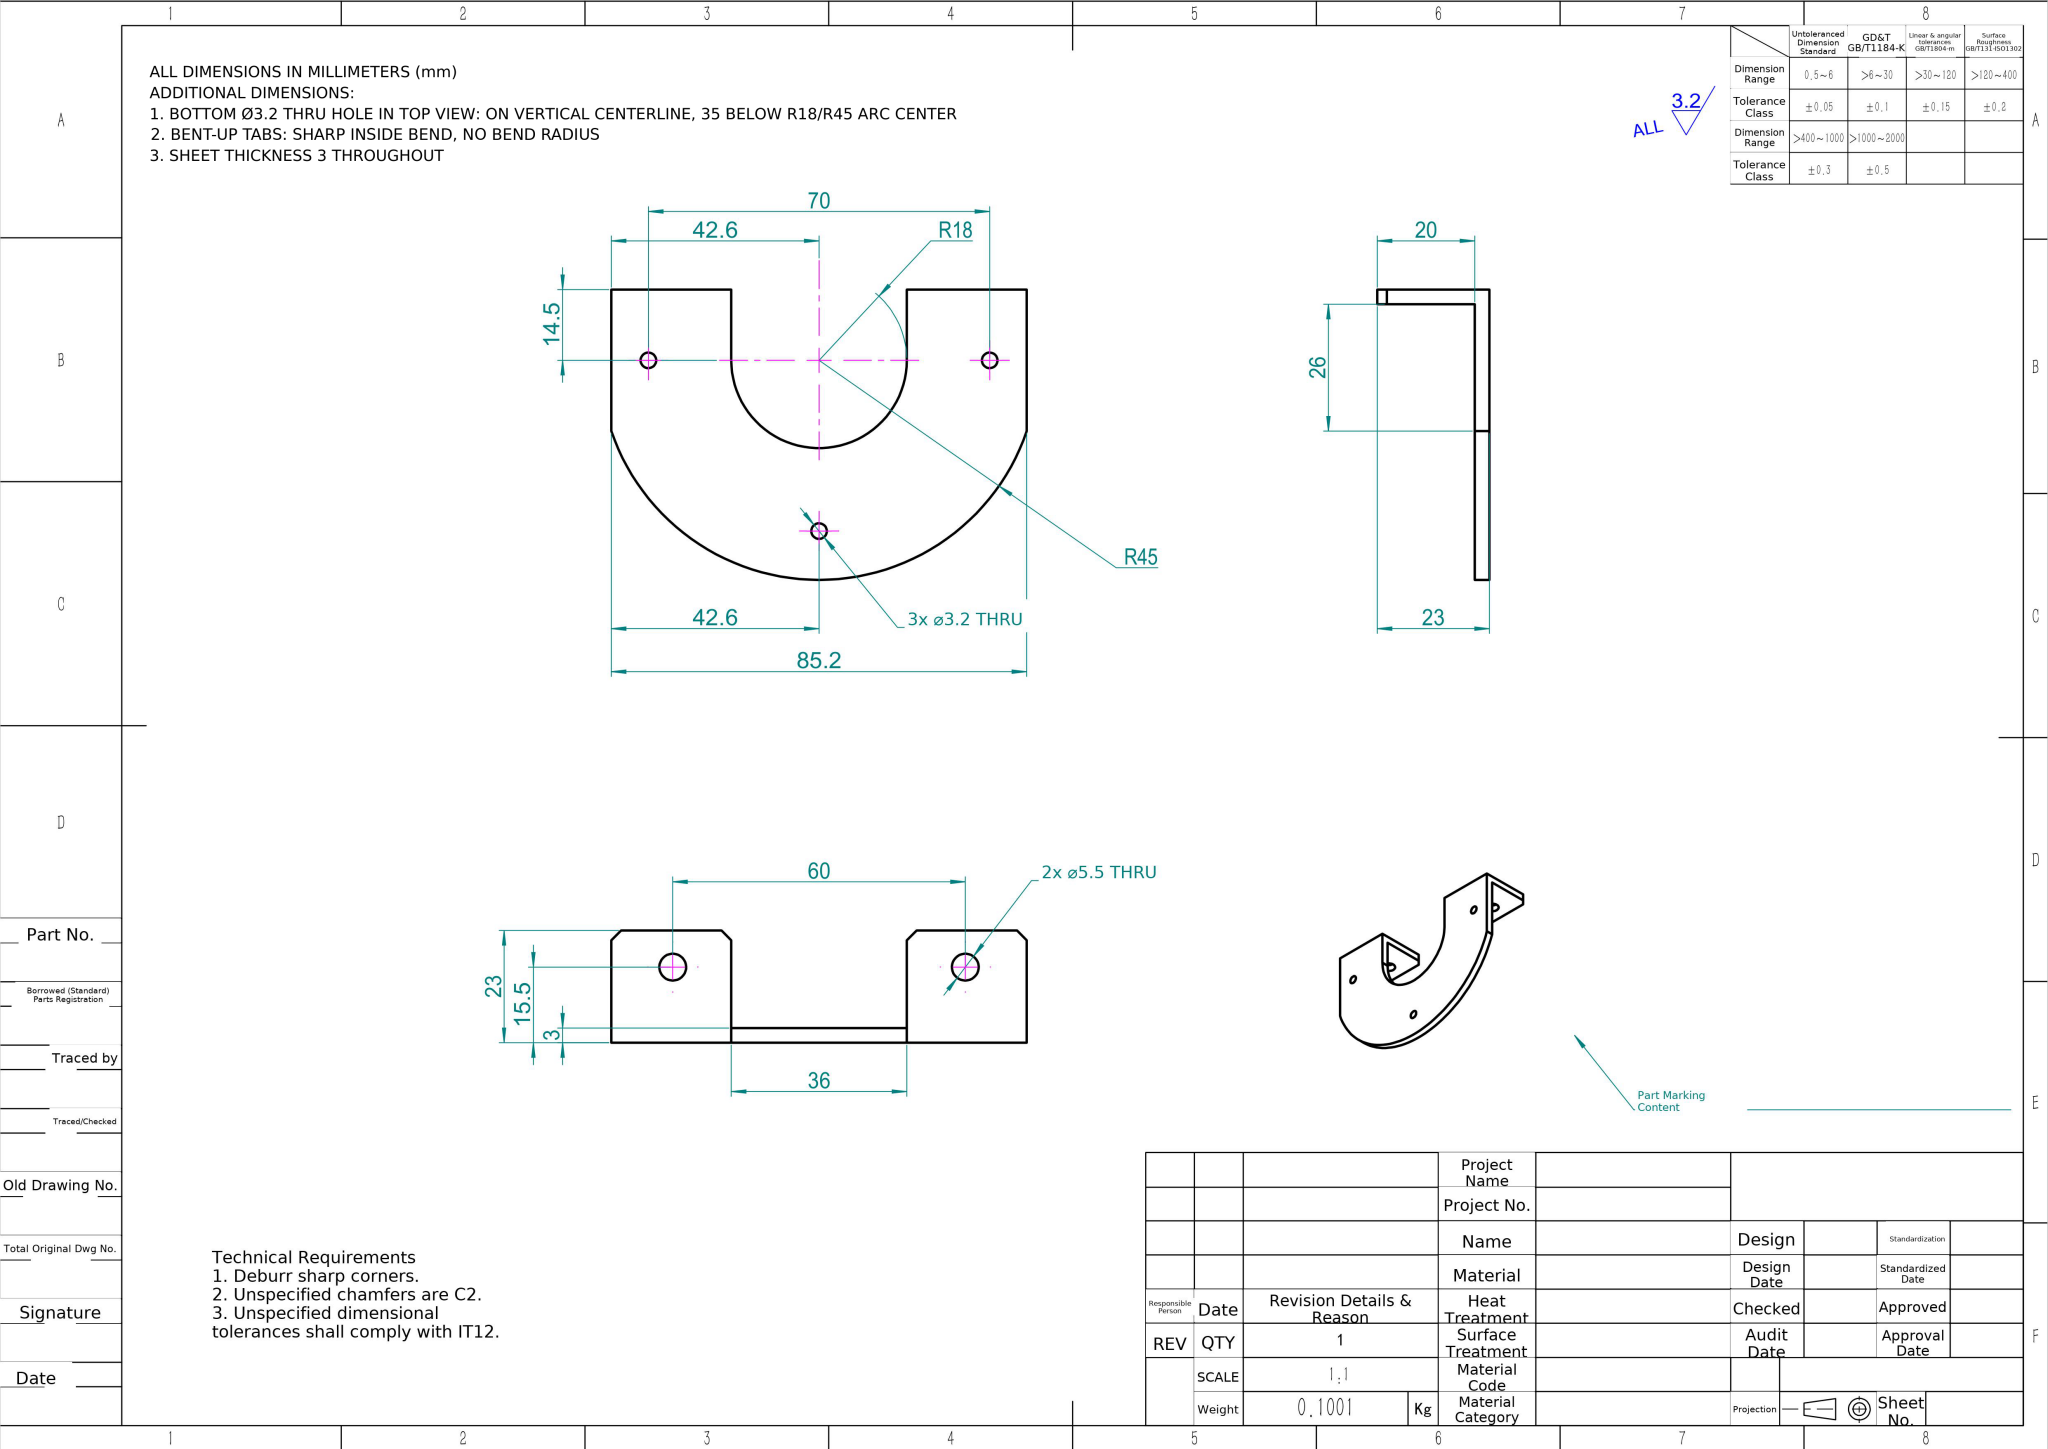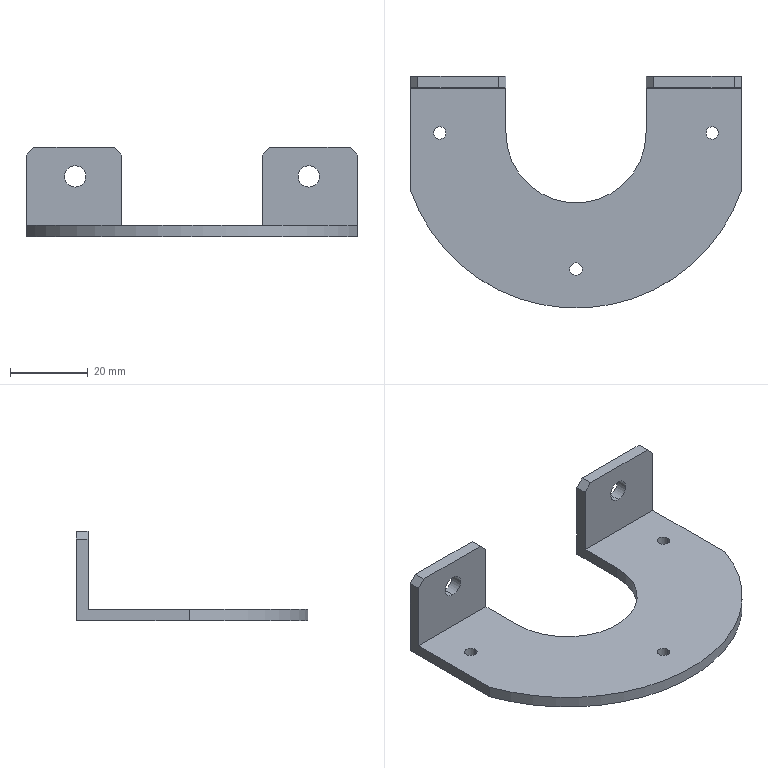Part | NX | mm | 1 solid | 28 faces | box 85.2 x 59.5 x 23 mm | volume 12729 mm3 | plane 16 | cylinder 12 | commonest cylinder face diameters 3.2 x6 5.5 x4 90 x1 36 x1
STEP:
#1=CARTESIAN_POINT('',(-36.6,0.,-0.));
#2=VERTEX_POINT('',#1);
#3=CARTESIAN_POINT('',(-33.4,0.,-0.));
#4=VERTEX_POINT('',#3);
#5=CARTESIAN_POINT('',(-35.,0.,-0.));
#6=DIRECTION('',(-0.,-0.,1.));
#7=DIRECTION('',(1.,0.,0.));
#8=AXIS2_PLACEMENT_3D('',#5,#6,#7);
#9=CIRCLE('',#8,1.6);
#10=EDGE_CURVE('',#2,#4,#9,.T.);
#11=ORIENTED_EDGE('',*,*,#10,.F.);
#12=CARTESIAN_POINT('',(-36.6,0.,3.));
#13=VERTEX_POINT('',#12);
#14=CARTESIAN_POINT('',(-36.6,0.,-0.));
#15=DIRECTION('',(-0.,-0.,1.));
#16=VECTOR('',#15,1000.);
#17=LINE('',#14,#16);
#18=EDGE_CURVE('',#2,#13,#17,.T.);
#19=ORIENTED_EDGE('',*,*,#18,.T.);
#20=CARTESIAN_POINT('',(-33.4,0.,3.));
#21=VERTEX_POINT('',#20);
#22=CARTESIAN_POINT('',(-35.,0.,3.));
#23=DIRECTION('',(-0.,-0.,1.));
#24=DIRECTION('',(1.,0.,0.));
#25=AXIS2_PLACEMENT_3D('',#22,#23,#24);
#26=CIRCLE('',#25,1.6);
#27=EDGE_CURVE('',#13,#21,#26,.T.);
#28=ORIENTED_EDGE('',*,*,#27,.T.);
#29=CARTESIAN_POINT('',(-33.4,0.,-0.));
#30=DIRECTION('',(-0.,-0.,1.));
#31=VECTOR('',#30,1000.);
#32=LINE('',#29,#31);
#33=EDGE_CURVE('',#4,#21,#32,.T.);
#34=ORIENTED_EDGE('',*,*,#33,.F.);
#35=EDGE_LOOP('',(#11,#19,#28,#34));
#36=FACE_OUTER_BOUND('',#35,.T.);
#37=CARTESIAN_POINT('',(-35.,0.,-0.));
#38=DIRECTION('',(-0.,-0.,1.));
#39=DIRECTION('',(1.,0.,0.));
#40=AXIS2_PLACEMENT_3D('',#37,#38,#39);
#41=CYLINDRICAL_SURFACE('',#40,1.6);
#42=ADVANCED_FACE('',(#36),#41,.F.);
#43=CARTESIAN_POINT('',(-1.6,-35.,-0.));
#44=VERTEX_POINT('',#43);
#45=CARTESIAN_POINT('',(1.6,-35.,0.));
#46=VERTEX_POINT('',#45);
#47=CARTESIAN_POINT('',(0.,-35.,0.));
#48=DIRECTION('',(-0.,-0.,1.));
#49=DIRECTION('',(1.,0.,0.));
#50=AXIS2_PLACEMENT_3D('',#47,#48,#49);
#51=CIRCLE('',#50,1.6);
#52=EDGE_CURVE('',#44,#46,#51,.T.);
#53=ORIENTED_EDGE('',*,*,#52,.F.);
#54=CARTESIAN_POINT('',(-1.6,-35.,3.));
#55=VERTEX_POINT('',#54);
#56=CARTESIAN_POINT('',(-1.6,-35.,-0.));
#57=DIRECTION('',(-0.,-0.,1.));
#58=VECTOR('',#57,1000.);
#59=LINE('',#56,#58);
#60=EDGE_CURVE('',#44,#55,#59,.T.);
#61=ORIENTED_EDGE('',*,*,#60,.T.);
#62=CARTESIAN_POINT('',(1.6,-35.,3.));
#63=VERTEX_POINT('',#62);
#64=CARTESIAN_POINT('',(-0.,-35.,3.));
#65=DIRECTION('',(-0.,-0.,1.));
#66=DIRECTION('',(1.,0.,0.));
#67=AXIS2_PLACEMENT_3D('',#64,#65,#66);
#68=CIRCLE('',#67,1.6);
#69=EDGE_CURVE('',#55,#63,#68,.T.);
#70=ORIENTED_EDGE('',*,*,#69,.T.);
#71=CARTESIAN_POINT('',(1.6,-35.,0.));
#72=DIRECTION('',(-0.,-0.,1.));
#73=VECTOR('',#72,1000.);
#74=LINE('',#71,#73);
#75=EDGE_CURVE('',#46,#63,#74,.T.);
#76=ORIENTED_EDGE('',*,*,#75,.F.);
#77=EDGE_LOOP('',(#53,#61,#70,#76));
#78=FACE_OUTER_BOUND('',#77,.T.);
#79=CARTESIAN_POINT('',(0.,-35.,0.));
#80=DIRECTION('',(-0.,-0.,1.));
#81=DIRECTION('',(1.,0.,0.));
#82=AXIS2_PLACEMENT_3D('',#79,#80,#81);
#83=CYLINDRICAL_SURFACE('',#82,1.6);
#84=ADVANCED_FACE('',(#78),#83,.F.);
#85=CARTESIAN_POINT('',(33.4,0.,-0.));
#86=VERTEX_POINT('',#85);
#87=CARTESIAN_POINT('',(36.6,0.,-0.));
#88=VERTEX_POINT('',#87);
#89=CARTESIAN_POINT('',(35.,0.,-0.));
#90=DIRECTION('',(-0.,-0.,1.));
#91=DIRECTION('',(1.,0.,0.));
#92=AXIS2_PLACEMENT_3D('',#89,#90,#91);
#93=CIRCLE('',#92,1.6);
#94=EDGE_CURVE('',#86,#88,#93,.T.);
#95=ORIENTED_EDGE('',*,*,#94,.F.);
#96=CARTESIAN_POINT('',(33.4,0.,3.));
#97=VERTEX_POINT('',#96);
#98=CARTESIAN_POINT('',(33.4,0.,-0.));
#99=DIRECTION('',(-0.,-0.,1.));
#100=VECTOR('',#99,1000.);
#101=LINE('',#98,#100);
#102=EDGE_CURVE('',#86,#97,#101,.T.);
#103=ORIENTED_EDGE('',*,*,#102,.T.);
#104=CARTESIAN_POINT('',(36.6,0.,3.));
#105=VERTEX_POINT('',#104);
#106=CARTESIAN_POINT('',(35.,0.,3.));
#107=DIRECTION('',(-0.,-0.,1.));
#108=DIRECTION('',(1.,0.,0.));
#109=AXIS2_PLACEMENT_3D('',#106,#107,#108);
#110=CIRCLE('',#109,1.6);
#111=EDGE_CURVE('',#97,#105,#110,.T.);
#112=ORIENTED_EDGE('',*,*,#111,.T.);
#113=CARTESIAN_POINT('',(36.6,0.,-0.));
#114=DIRECTION('',(-0.,-0.,1.));
#115=VECTOR('',#114,1000.);
#116=LINE('',#113,#115);
#117=EDGE_CURVE('',#88,#105,#116,.T.);
#118=ORIENTED_EDGE('',*,*,#117,.F.);
#119=EDGE_LOOP('',(#95,#103,#112,#118));
#120=FACE_OUTER_BOUND('',#119,.T.);
#121=CARTESIAN_POINT('',(35.,0.,-0.));
#122=DIRECTION('',(-0.,-0.,1.));
#123=DIRECTION('',(1.,0.,0.));
#124=AXIS2_PLACEMENT_3D('',#121,#122,#123);
#125=CYLINDRICAL_SURFACE('',#124,1.6);
#126=ADVANCED_FACE('',(#120),#125,.F.);
#127=CARTESIAN_POINT('',(-30.,14.5,18.25));
#128=VERTEX_POINT('',#127);
#129=CARTESIAN_POINT('',(-30.,14.5,12.75));
#130=VERTEX_POINT('',#129);
#131=CARTESIAN_POINT('',(-30.,14.5,15.5));
#132=DIRECTION('',(-0.,-1.,0.));
#133=DIRECTION('',(0.,0.,-1.));
#134=AXIS2_PLACEMENT_3D('',#131,#132,#133);
#135=CIRCLE('',#134,2.75);
#136=EDGE_CURVE('',#128,#130,#135,.T.);
#137=ORIENTED_EDGE('',*,*,#136,.F.);
#138=CARTESIAN_POINT('',(-30.,11.5,18.25));
#139=VERTEX_POINT('',#138);
#140=CARTESIAN_POINT('',(-30.,14.5,18.25));
#141=DIRECTION('',(-0.,-1.,0.));
#142=VECTOR('',#141,1000.);
#143=LINE('',#140,#142);
#144=EDGE_CURVE('',#128,#139,#143,.T.);
#145=ORIENTED_EDGE('',*,*,#144,.T.);
#146=CARTESIAN_POINT('',(-30.,11.5,12.75));
#147=VERTEX_POINT('',#146);
#148=CARTESIAN_POINT('',(-30.,11.5,15.5));
#149=DIRECTION('',(-0.,-1.,0.));
#150=DIRECTION('',(0.,0.,-1.));
#151=AXIS2_PLACEMENT_3D('',#148,#149,#150);
#152=CIRCLE('',#151,2.75);
#153=EDGE_CURVE('',#139,#147,#152,.T.);
#154=ORIENTED_EDGE('',*,*,#153,.T.);
#155=CARTESIAN_POINT('',(-30.,14.5,12.75));
#156=DIRECTION('',(-0.,-1.,0.));
#157=VECTOR('',#156,1000.);
#158=LINE('',#155,#157);
#159=EDGE_CURVE('',#130,#147,#158,.T.);
#160=ORIENTED_EDGE('',*,*,#159,.F.);
#161=EDGE_LOOP('',(#137,#145,#154,#160));
#162=FACE_OUTER_BOUND('',#161,.T.);
#163=CARTESIAN_POINT('',(-30.,14.5,15.5));
#164=DIRECTION('',(-0.,-1.,0.));
#165=DIRECTION('',(0.,0.,-1.));
#166=AXIS2_PLACEMENT_3D('',#163,#164,#165);
#167=CYLINDRICAL_SURFACE('',#166,2.75);
#168=ADVANCED_FACE('',(#162),#167,.F.);
#169=CARTESIAN_POINT('',(30.,14.5,18.25));
#170=VERTEX_POINT('',#169);
#171=CARTESIAN_POINT('',(30.,14.5,12.75));
#172=VERTEX_POINT('',#171);
#173=CARTESIAN_POINT('',(30.,14.5,15.5));
#174=DIRECTION('',(-0.,-1.,0.));
#175=DIRECTION('',(0.,0.,-1.));
#176=AXIS2_PLACEMENT_3D('',#173,#174,#175);
#177=CIRCLE('',#176,2.75);
#178=EDGE_CURVE('',#170,#172,#177,.T.);
#179=ORIENTED_EDGE('',*,*,#178,.F.);
#180=CARTESIAN_POINT('',(30.,11.5,18.25));
#181=VERTEX_POINT('',#180);
#182=CARTESIAN_POINT('',(30.,14.5,18.25));
#183=DIRECTION('',(-0.,-1.,0.));
#184=VECTOR('',#183,1000.);
#185=LINE('',#182,#184);
#186=EDGE_CURVE('',#170,#181,#185,.T.);
#187=ORIENTED_EDGE('',*,*,#186,.T.);
#188=CARTESIAN_POINT('',(30.,11.5,12.75));
#189=VERTEX_POINT('',#188);
#190=CARTESIAN_POINT('',(30.,11.5,15.5));
#191=DIRECTION('',(-0.,-1.,0.));
#192=DIRECTION('',(0.,0.,-1.));
#193=AXIS2_PLACEMENT_3D('',#190,#191,#192);
#194=CIRCLE('',#193,2.75);
#195=EDGE_CURVE('',#181,#189,#194,.T.);
#196=ORIENTED_EDGE('',*,*,#195,.T.);
#197=CARTESIAN_POINT('',(30.,14.5,12.75));
#198=DIRECTION('',(-0.,-1.,0.));
#199=VECTOR('',#198,1000.);
#200=LINE('',#197,#199);
#201=EDGE_CURVE('',#172,#189,#200,.T.);
#202=ORIENTED_EDGE('',*,*,#201,.F.);
#203=EDGE_LOOP('',(#179,#187,#196,#202));
#204=FACE_OUTER_BOUND('',#203,.T.);
#205=CARTESIAN_POINT('',(30.,14.5,15.5));
#206=DIRECTION('',(-0.,-1.,0.));
#207=DIRECTION('',(0.,0.,-1.));
#208=AXIS2_PLACEMENT_3D('',#205,#206,#207);
#209=CYLINDRICAL_SURFACE('',#208,2.75);
#210=ADVANCED_FACE('',(#204),#209,.F.);
#211=CARTESIAN_POINT('',(-35.,0.,3.));
#212=DIRECTION('',(-0.,-0.,1.));
#213=DIRECTION('',(1.,0.,0.));
#214=AXIS2_PLACEMENT_3D('',#211,#212,#213);
#215=CIRCLE('',#214,1.6);
#216=EDGE_CURVE('',#21,#13,#215,.T.);
#217=ORIENTED_EDGE('',*,*,#216,.F.);
#218=ORIENTED_EDGE('',*,*,#27,.F.);
#219=EDGE_LOOP('',(#217,#218));
#220=FACE_BOUND('',#219,.T.);
#221=CARTESIAN_POINT('',(-0.,-35.,3.));
#222=DIRECTION('',(-0.,-0.,1.));
#223=DIRECTION('',(1.,0.,0.));
#224=AXIS2_PLACEMENT_3D('',#221,#222,#223);
#225=CIRCLE('',#224,1.6);
#226=EDGE_CURVE('',#63,#55,#225,.T.);
#227=ORIENTED_EDGE('',*,*,#226,.F.);
#228=ORIENTED_EDGE('',*,*,#69,.F.);
#229=EDGE_LOOP('',(#227,#228));
#230=FACE_BOUND('',#229,.T.);
#231=CARTESIAN_POINT('',(35.,0.,3.));
#232=DIRECTION('',(-0.,-0.,1.));
#233=DIRECTION('',(1.,0.,0.));
#234=AXIS2_PLACEMENT_3D('',#231,#232,#233);
#235=CIRCLE('',#234,1.6);
#236=EDGE_CURVE('',#105,#97,#235,.T.);
#237=ORIENTED_EDGE('',*,*,#236,.F.);
#238=ORIENTED_EDGE('',*,*,#111,.F.);
#239=EDGE_LOOP('',(#237,#238));
#240=FACE_BOUND('',#239,.T.);
#241=CARTESIAN_POINT('',(-42.6,11.5,3.));
#242=VERTEX_POINT('',#241);
#243=CARTESIAN_POINT('',(-18.,11.5,3.));
#244=VERTEX_POINT('',#243);
#245=CARTESIAN_POINT('',(-42.6,11.5,3.));
#246=DIRECTION('',(1.,0.,0.));
#247=VECTOR('',#246,1000.);
#248=LINE('',#245,#247);
#249=EDGE_CURVE('',#242,#244,#248,.T.);
#250=ORIENTED_EDGE('',*,*,#249,.F.);
#251=CARTESIAN_POINT('',(-42.6,-14.5,3.));
#252=VERTEX_POINT('',#251);
#253=CARTESIAN_POINT('',(-42.6,14.5,3.));
#254=DIRECTION('',(-0.,-1.,0.));
#255=VECTOR('',#254,1000.);
#256=LINE('',#253,#255);
#257=EDGE_CURVE('',#242,#252,#256,.T.);
#258=ORIENTED_EDGE('',*,*,#257,.T.);
#259=CARTESIAN_POINT('',(42.6,-14.5,3.));
#260=VERTEX_POINT('',#259);
#261=CARTESIAN_POINT('',(-0.,0.,3.));
#262=DIRECTION('',(-0.,-0.,1.));
#263=DIRECTION('',(1.,0.,0.));
#264=AXIS2_PLACEMENT_3D('',#261,#262,#263);
#265=CIRCLE('',#264,45.);
#266=EDGE_CURVE('',#252,#260,#265,.T.);
#267=ORIENTED_EDGE('',*,*,#266,.T.);
#268=CARTESIAN_POINT('',(42.6,11.5,3.));
#269=VERTEX_POINT('',#268);
#270=CARTESIAN_POINT('',(42.6,14.5,3.));
#271=DIRECTION('',(-0.,1.,-0.));
#272=VECTOR('',#271,1000.);
#273=LINE('',#270,#272);
#274=EDGE_CURVE('',#260,#269,#273,.T.);
#275=ORIENTED_EDGE('',*,*,#274,.T.);
#276=CARTESIAN_POINT('',(18.,11.5,3.));
#277=VERTEX_POINT('',#276);
#278=CARTESIAN_POINT('',(18.,11.5,3.));
#279=DIRECTION('',(1.,0.,0.));
#280=VECTOR('',#279,1000.);
#281=LINE('',#278,#280);
#282=EDGE_CURVE('',#277,#269,#281,.T.);
#283=ORIENTED_EDGE('',*,*,#282,.F.);
#284=CARTESIAN_POINT('',(18.,-0.,3.));
#285=VERTEX_POINT('',#284);
#286=CARTESIAN_POINT('',(18.,-0.,3.));
#287=DIRECTION('',(0.,1.,-0.));
#288=VECTOR('',#287,1000.);
#289=LINE('',#286,#288);
#290=EDGE_CURVE('',#285,#277,#289,.T.);
#291=ORIENTED_EDGE('',*,*,#290,.F.);
#292=CARTESIAN_POINT('',(-18.,-0.,3.));
#293=VERTEX_POINT('',#292);
#294=CARTESIAN_POINT('',(-0.,0.,3.));
#295=DIRECTION('',(-0.,-0.,1.));
#296=DIRECTION('',(1.,0.,0.));
#297=AXIS2_PLACEMENT_3D('',#294,#295,#296);
#298=CIRCLE('',#297,18.);
#299=EDGE_CURVE('',#293,#285,#298,.T.);
#300=ORIENTED_EDGE('',*,*,#299,.F.);
#301=CARTESIAN_POINT('',(-18.,-0.,3.));
#302=DIRECTION('',(-0.,-1.,0.));
#303=VECTOR('',#302,1000.);
#304=LINE('',#301,#303);
#305=EDGE_CURVE('',#244,#293,#304,.T.);
#306=ORIENTED_EDGE('',*,*,#305,.F.);
#307=EDGE_LOOP('',(#250,#258,#267,#275,#283,#291,#300,#306));
#308=FACE_OUTER_BOUND('',#307,.T.);
#309=CARTESIAN_POINT('',(-0.,0.,3.));
#310=DIRECTION('',(-0.,-0.,1.));
#311=DIRECTION('',(1.,0.,0.));
#312=AXIS2_PLACEMENT_3D('',#309,#310,#311);
#313=PLANE('',#312);
#314=ADVANCED_FACE('',(#220,#230,#240,#308),#313,.T.);
#315=CARTESIAN_POINT('',(-35.,0.,-0.));
#316=DIRECTION('',(-0.,-0.,1.));
#317=DIRECTION('',(1.,0.,0.));
#318=AXIS2_PLACEMENT_3D('',#315,#316,#317);
#319=CIRCLE('',#318,1.6);
#320=EDGE_CURVE('',#4,#2,#319,.T.);
#321=ORIENTED_EDGE('',*,*,#320,.T.);
#322=ORIENTED_EDGE('',*,*,#10,.T.);
#323=EDGE_LOOP('',(#321,#322));
#324=FACE_BOUND('',#323,.T.);
#325=CARTESIAN_POINT('',(0.,-35.,0.));
#326=DIRECTION('',(-0.,-0.,1.));
#327=DIRECTION('',(1.,0.,0.));
#328=AXIS2_PLACEMENT_3D('',#325,#326,#327);
#329=CIRCLE('',#328,1.6);
#330=EDGE_CURVE('',#46,#44,#329,.T.);
#331=ORIENTED_EDGE('',*,*,#330,.T.);
#332=ORIENTED_EDGE('',*,*,#52,.T.);
#333=EDGE_LOOP('',(#331,#332));
#334=FACE_BOUND('',#333,.T.);
#335=CARTESIAN_POINT('',(35.,0.,-0.));
#336=DIRECTION('',(-0.,-0.,1.));
#337=DIRECTION('',(1.,0.,0.));
#338=AXIS2_PLACEMENT_3D('',#335,#336,#337);
#339=CIRCLE('',#338,1.6);
#340=EDGE_CURVE('',#88,#86,#339,.T.);
#341=ORIENTED_EDGE('',*,*,#340,.T.);
#342=ORIENTED_EDGE('',*,*,#94,.T.);
#343=EDGE_LOOP('',(#341,#342));
#344=FACE_BOUND('',#343,.T.);
#345=CARTESIAN_POINT('',(-42.6,14.5,-0.));
#346=VERTEX_POINT('',#345);
#347=CARTESIAN_POINT('',(-42.6,-14.5,-0.));
#348=VERTEX_POINT('',#347);
#349=CARTESIAN_POINT('',(-42.6,14.5,-0.));
#350=DIRECTION('',(-0.,-1.,0.));
#351=VECTOR('',#350,1000.);
#352=LINE('',#349,#351);
#353=EDGE_CURVE('',#346,#348,#352,.T.);
#354=ORIENTED_EDGE('',*,*,#353,.F.);
#355=CARTESIAN_POINT('',(-18.,14.5,-0.));
#356=VERTEX_POINT('',#355);
#357=CARTESIAN_POINT('',(-42.6,14.5,-0.));
#358=DIRECTION('',(1.,0.,0.));
#359=VECTOR('',#358,1000.);
#360=LINE('',#357,#359);
#361=EDGE_CURVE('',#346,#356,#360,.T.);
#362=ORIENTED_EDGE('',*,*,#361,.T.);
#363=CARTESIAN_POINT('',(-18.,-0.,0.));
#364=VERTEX_POINT('',#363);
#365=CARTESIAN_POINT('',(-18.,-0.,0.));
#366=DIRECTION('',(-0.,-1.,0.));
#367=VECTOR('',#366,1000.);
#368=LINE('',#365,#367);
#369=EDGE_CURVE('',#356,#364,#368,.T.);
#370=ORIENTED_EDGE('',*,*,#369,.T.);
#371=CARTESIAN_POINT('',(18.,-0.,-0.));
#372=VERTEX_POINT('',#371);
#373=CARTESIAN_POINT('',(0.,0.,0.));
#374=DIRECTION('',(-0.,-0.,1.));
#375=DIRECTION('',(1.,0.,0.));
#376=AXIS2_PLACEMENT_3D('',#373,#374,#375);
#377=CIRCLE('',#376,18.);
#378=EDGE_CURVE('',#364,#372,#377,.T.);
#379=ORIENTED_EDGE('',*,*,#378,.T.);
#380=CARTESIAN_POINT('',(18.,14.5,-0.));
#381=VERTEX_POINT('',#380);
#382=CARTESIAN_POINT('',(18.,-0.,-0.));
#383=DIRECTION('',(0.,1.,-0.));
#384=VECTOR('',#383,1000.);
#385=LINE('',#382,#384);
#386=EDGE_CURVE('',#372,#381,#385,.T.);
#387=ORIENTED_EDGE('',*,*,#386,.T.);
#388=CARTESIAN_POINT('',(42.6,14.5,-0.));
#389=VERTEX_POINT('',#388);
#390=CARTESIAN_POINT('',(-42.6,14.5,-0.));
#391=DIRECTION('',(1.,0.,0.));
#392=VECTOR('',#391,1000.);
#393=LINE('',#390,#392);
#394=EDGE_CURVE('',#381,#389,#393,.T.);
#395=ORIENTED_EDGE('',*,*,#394,.T.);
#396=CARTESIAN_POINT('',(42.6,-14.5,-0.));
#397=VERTEX_POINT('',#396);
#398=CARTESIAN_POINT('',(42.6,14.5,-0.));
#399=DIRECTION('',(-0.,1.,-0.));
#400=VECTOR('',#399,1000.);
#401=LINE('',#398,#400);
#402=EDGE_CURVE('',#397,#389,#401,.T.);
#403=ORIENTED_EDGE('',*,*,#402,.F.);
#404=CARTESIAN_POINT('',(0.,0.,0.));
#405=DIRECTION('',(-0.,-0.,1.));
#406=DIRECTION('',(1.,0.,0.));
#407=AXIS2_PLACEMENT_3D('',#404,#405,#406);
#408=CIRCLE('',#407,45.);
#409=EDGE_CURVE('',#348,#397,#408,.T.);
#410=ORIENTED_EDGE('',*,*,#409,.F.);
#411=EDGE_LOOP('',(#354,#362,#370,#379,#387,#395,#403,#410));
#412=FACE_OUTER_BOUND('',#411,.T.);
#413=CARTESIAN_POINT('',(0.,0.,0.));
#414=DIRECTION('',(-0.,-0.,1.));
#415=DIRECTION('',(1.,0.,0.));
#416=AXIS2_PLACEMENT_3D('',#413,#414,#415);
#417=PLANE('',#416);
#418=ADVANCED_FACE('',(#324,#334,#344,#412),#417,.F.);
#419=CARTESIAN_POINT('',(-42.6,-14.5,3.));
#420=DIRECTION('',(-0.,-0.,1.));
#421=VECTOR('',#420,1000.);
#422=LINE('',#419,#421);
#423=EDGE_CURVE('',#348,#252,#422,.T.);
#424=ORIENTED_EDGE('',*,*,#423,.F.);
#425=ORIENTED_EDGE('',*,*,#409,.T.);
#426=CARTESIAN_POINT('',(42.6,-14.5,3.));
#427=DIRECTION('',(0.,0.,-1.));
#428=VECTOR('',#427,1000.);
#429=LINE('',#426,#428);
#430=EDGE_CURVE('',#260,#397,#429,.T.);
#431=ORIENTED_EDGE('',*,*,#430,.F.);
#432=ORIENTED_EDGE('',*,*,#266,.F.);
#433=EDGE_LOOP('',(#424,#425,#431,#432));
#434=FACE_OUTER_BOUND('',#433,.T.);
#435=CARTESIAN_POINT('',(-0.,0.,3.));
#436=DIRECTION('',(0.,0.,-1.));
#437=DIRECTION('',(-1.,-0.,-0.));
#438=AXIS2_PLACEMENT_3D('',#435,#436,#437);
#439=CYLINDRICAL_SURFACE('',#438,45.);
#440=ADVANCED_FACE('',(#434),#439,.T.);
#441=CARTESIAN_POINT('',(-18.,-0.,0.));
#442=DIRECTION('',(-0.,-0.,1.));
#443=VECTOR('',#442,1000.);
#444=LINE('',#441,#443);
#445=EDGE_CURVE('',#364,#293,#444,.T.);
#446=ORIENTED_EDGE('',*,*,#445,.T.);
#447=ORIENTED_EDGE('',*,*,#299,.T.);
#448=CARTESIAN_POINT('',(18.,-0.,-0.));
#449=DIRECTION('',(-0.,-0.,1.));
#450=VECTOR('',#449,1000.);
#451=LINE('',#448,#450);
#452=EDGE_CURVE('',#372,#285,#451,.T.);
#453=ORIENTED_EDGE('',*,*,#452,.F.);
#454=ORIENTED_EDGE('',*,*,#378,.F.);
#455=EDGE_LOOP('',(#446,#447,#453,#454));
#456=FACE_OUTER_BOUND('',#455,.T.);
#457=CARTESIAN_POINT('',(-0.,0.,3.));
#458=DIRECTION('',(0.,0.,-1.));
#459=DIRECTION('',(-1.,-0.,-0.));
#460=AXIS2_PLACEMENT_3D('',#457,#458,#459);
#461=CYLINDRICAL_SURFACE('',#460,18.);
#462=ADVANCED_FACE('',(#456),#461,.F.);
#463=CARTESIAN_POINT('',(30.,14.5,15.5));
#464=DIRECTION('',(-0.,-1.,0.));
#465=DIRECTION('',(0.,0.,-1.));
#466=AXIS2_PLACEMENT_3D('',#463,#464,#465);
#467=CIRCLE('',#466,2.75);
#468=EDGE_CURVE('',#172,#170,#467,.T.);
#469=ORIENTED_EDGE('',*,*,#468,.T.);
#470=ORIENTED_EDGE('',*,*,#178,.T.);
#471=EDGE_LOOP('',(#469,#470));
#472=FACE_BOUND('',#471,.T.);
#473=CARTESIAN_POINT('',(40.6,14.5,23.));
#474=VERTEX_POINT('',#473);
#475=CARTESIAN_POINT('',(20.,14.5,23.));
#476=VERTEX_POINT('',#475);
#477=CARTESIAN_POINT('',(18.,14.5,23.));
#478=DIRECTION('',(-1.,-0.,-0.));
#479=VECTOR('',#478,1000.);
#480=LINE('',#477,#479);
#481=EDGE_CURVE('',#474,#476,#480,.T.);
#482=ORIENTED_EDGE('',*,*,#481,.F.);
#483=CARTESIAN_POINT('',(42.6,14.5,21.));
#484=VERTEX_POINT('',#483);
#485=CARTESIAN_POINT('',(40.6,14.5,23.));
#486=DIRECTION('',(0.7071,0.,-0.7071));
#487=VECTOR('',#486,1000.);
#488=LINE('',#485,#487);
#489=EDGE_CURVE('',#474,#484,#488,.T.);
#490=ORIENTED_EDGE('',*,*,#489,.T.);
#491=CARTESIAN_POINT('',(42.6,14.5,-0.));
#492=DIRECTION('',(-0.,-0.,1.));
#493=VECTOR('',#492,1000.);
#494=LINE('',#491,#493);
#495=EDGE_CURVE('',#389,#484,#494,.T.);
#496=ORIENTED_EDGE('',*,*,#495,.F.);
#497=ORIENTED_EDGE('',*,*,#394,.F.);
#498=CARTESIAN_POINT('',(18.,14.5,21.));
#499=VERTEX_POINT('',#498);
#500=CARTESIAN_POINT('',(18.,14.5,-0.));
#501=DIRECTION('',(-0.,-0.,1.));
#502=VECTOR('',#501,1000.);
#503=LINE('',#500,#502);
#504=EDGE_CURVE('',#381,#499,#503,.T.);
#505=ORIENTED_EDGE('',*,*,#504,.T.);
#506=CARTESIAN_POINT('',(20.,14.5,23.));
#507=DIRECTION('',(0.7071,-0.,0.7071));
#508=VECTOR('',#507,1000.);
#509=LINE('',#506,#508);
#510=EDGE_CURVE('',#499,#476,#509,.T.);
#511=ORIENTED_EDGE('',*,*,#510,.T.);
#512=EDGE_LOOP('',(#482,#490,#496,#497,#505,#511));
#513=FACE_OUTER_BOUND('',#512,.T.);
#514=CARTESIAN_POINT('',(-42.6,14.5,-0.));
#515=DIRECTION('',(-0.,-1.,-0.));
#516=DIRECTION('',(0.,0.,-1.));
#517=AXIS2_PLACEMENT_3D('',#514,#515,#516);
#518=PLANE('',#517);
#519=ADVANCED_FACE('',(#472,#513),#518,.F.);
#520=CARTESIAN_POINT('',(-30.,14.5,15.5));
#521=DIRECTION('',(-0.,-1.,0.));
#522=DIRECTION('',(0.,0.,-1.));
#523=AXIS2_PLACEMENT_3D('',#520,#521,#522);
#524=CIRCLE('',#523,2.75);
#525=EDGE_CURVE('',#130,#128,#524,.T.);
#526=ORIENTED_EDGE('',*,*,#525,.T.);
#527=ORIENTED_EDGE('',*,*,#136,.T.);
#528=EDGE_LOOP('',(#526,#527));
#529=FACE_BOUND('',#528,.T.);
#530=CARTESIAN_POINT('',(-20.,14.5,23.));
#531=VERTEX_POINT('',#530);
#532=CARTESIAN_POINT('',(-40.6,14.5,23.));
#533=VERTEX_POINT('',#532);
#534=CARTESIAN_POINT('',(-42.6,14.5,23.));
#535=DIRECTION('',(-1.,-0.,-0.));
#536=VECTOR('',#535,1000.);
#537=LINE('',#534,#536);
#538=EDGE_CURVE('',#531,#533,#537,.T.);
#539=ORIENTED_EDGE('',*,*,#538,.F.);
#540=CARTESIAN_POINT('',(-18.,14.5,21.));
#541=VERTEX_POINT('',#540);
#542=CARTESIAN_POINT('',(-20.,14.5,23.));
#543=DIRECTION('',(0.7071,0.,-0.7071));
#544=VECTOR('',#543,1000.);
#545=LINE('',#542,#544);
#546=EDGE_CURVE('',#531,#541,#545,.T.);
#547=ORIENTED_EDGE('',*,*,#546,.T.);
#548=CARTESIAN_POINT('',(-18.,14.5,-0.));
#549=DIRECTION('',(0.,0.,-1.));
#550=VECTOR('',#549,1000.);
#551=LINE('',#548,#550);
#552=EDGE_CURVE('',#541,#356,#551,.T.);
#553=ORIENTED_EDGE('',*,*,#552,.T.);
#554=ORIENTED_EDGE('',*,*,#361,.F.);
#555=CARTESIAN_POINT('',(-42.6,14.5,21.));
#556=VERTEX_POINT('',#555);
#557=CARTESIAN_POINT('',(-42.6,14.5,-0.));
#558=DIRECTION('',(-0.,-0.,1.));
#559=VECTOR('',#558,1000.);
#560=LINE('',#557,#559);
#561=EDGE_CURVE('',#346,#556,#560,.T.);
#562=ORIENTED_EDGE('',*,*,#561,.T.);
#563=CARTESIAN_POINT('',(-40.6,14.5,23.));
#564=DIRECTION('',(0.7071,-0.,0.7071));
#565=VECTOR('',#564,1000.);
#566=LINE('',#563,#565);
#567=EDGE_CURVE('',#556,#533,#566,.T.);
#568=ORIENTED_EDGE('',*,*,#567,.T.);
#569=EDGE_LOOP('',(#539,#547,#553,#554,#562,#568));
#570=FACE_OUTER_BOUND('',#569,.T.);
#571=CARTESIAN_POINT('',(-42.6,14.5,-0.));
#572=DIRECTION('',(-0.,-1.,-0.));
#573=DIRECTION('',(0.,0.,-1.));
#574=AXIS2_PLACEMENT_3D('',#571,#572,#573);
#575=PLANE('',#574);
#576=ADVANCED_FACE('',(#529,#570),#575,.F.);
#577=ORIENTED_EDGE('',*,*,#552,.F.);
#578=CARTESIAN_POINT('',(-18.,11.5,21.));
#579=VERTEX_POINT('',#578);
#580=CARTESIAN_POINT('',(-18.,11.5,21.));
#581=DIRECTION('',(-0.,-1.,0.));
#582=VECTOR('',#581,1000.);
#583=LINE('',#580,#582);
#584=EDGE_CURVE('',#541,#579,#583,.T.);
#585=ORIENTED_EDGE('',*,*,#584,.T.);
#586=CARTESIAN_POINT('',(-18.,11.5,23.));
#587=DIRECTION('',(0.,0.,-1.));
#588=VECTOR('',#587,1000.);
#589=LINE('',#586,#588);
#590=EDGE_CURVE('',#579,#244,#589,.T.);
#591=ORIENTED_EDGE('',*,*,#590,.T.);
#592=ORIENTED_EDGE('',*,*,#305,.T.);
#593=ORIENTED_EDGE('',*,*,#445,.F.);
#594=ORIENTED_EDGE('',*,*,#369,.F.);
#595=EDGE_LOOP('',(#577,#585,#591,#592,#593,#594));
#596=FACE_OUTER_BOUND('',#595,.T.);
#597=CARTESIAN_POINT('',(-18.,-0.,0.));
#598=DIRECTION('',(-1.,-0.,-0.));
#599=DIRECTION('',(-0.,-0.,1.));
#600=AXIS2_PLACEMENT_3D('',#597,#598,#599);
#601=PLANE('',#600);
#602=ADVANCED_FACE('',(#596),#601,.F.);
#603=CARTESIAN_POINT('',(18.,11.5,21.));
#604=VERTEX_POINT('',#603);
#605=CARTESIAN_POINT('',(18.,11.5,23.));
#606=DIRECTION('',(0.,0.,-1.));
#607=VECTOR('',#606,1000.);
#608=LINE('',#605,#607);
#609=EDGE_CURVE('',#604,#277,#608,.T.);
#610=ORIENTED_EDGE('',*,*,#609,.F.);
#611=CARTESIAN_POINT('',(18.,14.5,21.));
#612=DIRECTION('',(0.,1.,-0.));
#613=VECTOR('',#612,1000.);
#614=LINE('',#611,#613);
#615=EDGE_CURVE('',#604,#499,#614,.T.);
#616=ORIENTED_EDGE('',*,*,#615,.T.);
#617=ORIENTED_EDGE('',*,*,#504,.F.);
#618=ORIENTED_EDGE('',*,*,#386,.F.);
#619=ORIENTED_EDGE('',*,*,#452,.T.);
#620=ORIENTED_EDGE('',*,*,#290,.T.);
#621=EDGE_LOOP('',(#610,#616,#617,#618,#619,#620));
#622=FACE_OUTER_BOUND('',#621,.T.);
#623=CARTESIAN_POINT('',(18.,-0.,-0.));
#624=DIRECTION('',(1.,0.,0.));
#625=DIRECTION('',(0.,0.,-1.));
#626=AXIS2_PLACEMENT_3D('',#623,#624,#625);
#627=PLANE('',#626);
#628=ADVANCED_FACE('',(#622),#627,.F.);
#629=CARTESIAN_POINT('',(-42.6,11.5,21.));
#630=VERTEX_POINT('',#629);
#631=CARTESIAN_POINT('',(-42.6,11.5,23.));
#632=DIRECTION('',(0.,0.,-1.));
#633=VECTOR('',#632,1000.);
#634=LINE('',#631,#633);
#635=EDGE_CURVE('',#630,#242,#634,.T.);
#636=ORIENTED_EDGE('',*,*,#635,.F.);
#637=CARTESIAN_POINT('',(-42.6,14.5,21.));
#638=DIRECTION('',(0.,1.,-0.));
#639=VECTOR('',#638,1000.);
#640=LINE('',#637,#639);
#641=EDGE_CURVE('',#630,#556,#640,.T.);
#642=ORIENTED_EDGE('',*,*,#641,.T.);
#643=ORIENTED_EDGE('',*,*,#561,.F.);
#644=ORIENTED_EDGE('',*,*,#353,.T.);
#645=ORIENTED_EDGE('',*,*,#423,.T.);
#646=ORIENTED_EDGE('',*,*,#257,.F.);
#647=EDGE_LOOP('',(#636,#642,#643,#644,#645,#646));
#648=FACE_OUTER_BOUND('',#647,.T.);
#649=CARTESIAN_POINT('',(-42.6,14.5,23.));
#650=DIRECTION('',(1.,0.,0.));
#651=DIRECTION('',(0.,0.,-1.));
#652=AXIS2_PLACEMENT_3D('',#649,#650,#651);
#653=PLANE('',#652);
#654=ADVANCED_FACE('',(#648),#653,.F.);
#655=CARTESIAN_POINT('',(-30.,11.5,15.5));
#656=DIRECTION('',(-0.,-1.,0.));
#657=DIRECTION('',(0.,0.,-1.));
#658=AXIS2_PLACEMENT_3D('',#655,#656,#657);
#659=CIRCLE('',#658,2.75);
#660=EDGE_CURVE('',#147,#139,#659,.T.);
#661=ORIENTED_EDGE('',*,*,#660,.F.);
#662=ORIENTED_EDGE('',*,*,#153,.F.);
#663=EDGE_LOOP('',(#661,#662));
#664=FACE_BOUND('',#663,.T.);
#665=ORIENTED_EDGE('',*,*,#590,.F.);
#666=CARTESIAN_POINT('',(-20.,11.5,23.));
#667=VERTEX_POINT('',#666);
#668=CARTESIAN_POINT('',(-20.,11.5,23.));
#669=DIRECTION('',(-0.7071,-0.,0.7071));
#670=VECTOR('',#669,1000.);
#671=LINE('',#668,#670);
#672=EDGE_CURVE('',#579,#667,#671,.T.);
#673=ORIENTED_EDGE('',*,*,#672,.T.);
#674=CARTESIAN_POINT('',(-40.6,11.5,23.));
#675=VERTEX_POINT('',#674);
#676=CARTESIAN_POINT('',(-42.6,11.5,23.));
#677=DIRECTION('',(1.,0.,0.));
#678=VECTOR('',#677,1000.);
#679=LINE('',#676,#678);
#680=EDGE_CURVE('',#675,#667,#679,.T.);
#681=ORIENTED_EDGE('',*,*,#680,.F.);
#682=CARTESIAN_POINT('',(-40.6,11.5,23.));
#683=DIRECTION('',(-0.7071,0.,-0.7071));
#684=VECTOR('',#683,1000.);
#685=LINE('',#682,#684);
#686=EDGE_CURVE('',#675,#630,#685,.T.);
#687=ORIENTED_EDGE('',*,*,#686,.T.);
#688=ORIENTED_EDGE('',*,*,#635,.T.);
#689=ORIENTED_EDGE('',*,*,#249,.T.);
#690=EDGE_LOOP('',(#665,#673,#681,#687,#688,#689));
#691=FACE_OUTER_BOUND('',#690,.T.);
#692=CARTESIAN_POINT('',(-42.6,11.5,23.));
#693=DIRECTION('',(0.,1.,0.));
#694=DIRECTION('',(-0.,-0.,1.));
#695=AXIS2_PLACEMENT_3D('',#692,#693,#694);
#696=PLANE('',#695);
#697=ADVANCED_FACE('',(#664,#691),#696,.F.);
#698=ORIENTED_EDGE('',*,*,#680,.T.);
#699=CARTESIAN_POINT('',(-20.,14.5,23.));
#700=DIRECTION('',(0.,1.,-0.));
#701=VECTOR('',#700,1000.);
#702=LINE('',#699,#701);
#703=EDGE_CURVE('',#667,#531,#702,.T.);
#704=ORIENTED_EDGE('',*,*,#703,.T.);
#705=ORIENTED_EDGE('',*,*,#538,.T.);
#706=CARTESIAN_POINT('',(-40.6,11.5,23.));
#707=DIRECTION('',(-0.,-1.,0.));
#708=VECTOR('',#707,1000.);
#709=LINE('',#706,#708);
#710=EDGE_CURVE('',#533,#675,#709,.T.);
#711=ORIENTED_EDGE('',*,*,#710,.T.);
#712=EDGE_LOOP('',(#698,#704,#705,#711));
#713=FACE_OUTER_BOUND('',#712,.T.);
#714=CARTESIAN_POINT('',(-0.,0.,23.));
#715=DIRECTION('',(-0.,-0.,1.));
#716=DIRECTION('',(1.,0.,0.));
#717=AXIS2_PLACEMENT_3D('',#714,#715,#716);
#718=PLANE('',#717);
#719=ADVANCED_FACE('',(#713),#718,.T.);
#720=CARTESIAN_POINT('',(30.,11.5,15.5));
#721=DIRECTION('',(-0.,-1.,0.));
#722=DIRECTION('',(0.,0.,-1.));
#723=AXIS2_PLACEMENT_3D('',#720,#721,#722);
#724=CIRCLE('',#723,2.75);
#725=EDGE_CURVE('',#189,#181,#724,.T.);
#726=ORIENTED_EDGE('',*,*,#725,.F.);
#727=ORIENTED_EDGE('',*,*,#195,.F.);
#728=EDGE_LOOP('',(#726,#727));
#729=FACE_BOUND('',#728,.T.);
#730=CARTESIAN_POINT('',(42.6,11.5,21.));
#731=VERTEX_POINT('',#730);
#732=CARTESIAN_POINT('',(42.6,11.5,23.));
#733=DIRECTION('',(0.,0.,-1.));
#734=VECTOR('',#733,1000.);
#735=LINE('',#732,#734);
#736=EDGE_CURVE('',#731,#269,#735,.T.);
#737=ORIENTED_EDGE('',*,*,#736,.F.);
#738=CARTESIAN_POINT('',(40.6,11.5,23.));
#739=VERTEX_POINT('',#738);
#740=CARTESIAN_POINT('',(40.6,11.5,23.));
#741=DIRECTION('',(-0.7071,-0.,0.7071));
#742=VECTOR('',#741,1000.);
#743=LINE('',#740,#742);
#744=EDGE_CURVE('',#731,#739,#743,.T.);
#745=ORIENTED_EDGE('',*,*,#744,.T.);
#746=CARTESIAN_POINT('',(20.,11.5,23.));
#747=VERTEX_POINT('',#746);
#748=CARTESIAN_POINT('',(18.,11.5,23.));
#749=DIRECTION('',(1.,0.,0.));
#750=VECTOR('',#749,1000.);
#751=LINE('',#748,#750);
#752=EDGE_CURVE('',#747,#739,#751,.T.);
#753=ORIENTED_EDGE('',*,*,#752,.F.);
#754=CARTESIAN_POINT('',(20.,11.5,23.));
#755=DIRECTION('',(-0.7071,0.,-0.7071));
#756=VECTOR('',#755,1000.);
#757=LINE('',#754,#756);
#758=EDGE_CURVE('',#747,#604,#757,.T.);
#759=ORIENTED_EDGE('',*,*,#758,.T.);
#760=ORIENTED_EDGE('',*,*,#609,.T.);
#761=ORIENTED_EDGE('',*,*,#282,.T.);
#762=EDGE_LOOP('',(#737,#745,#753,#759,#760,#761));
#763=FACE_OUTER_BOUND('',#762,.T.);
#764=CARTESIAN_POINT('',(18.,11.5,23.));
#765=DIRECTION('',(0.,1.,0.));
#766=DIRECTION('',(-0.,-0.,1.));
#767=AXIS2_PLACEMENT_3D('',#764,#765,#766);
#768=PLANE('',#767);
#769=ADVANCED_FACE('',(#729,#763),#768,.F.);
#770=ORIENTED_EDGE('',*,*,#495,.T.);
#771=CARTESIAN_POINT('',(42.6,11.5,21.));
#772=DIRECTION('',(-0.,-1.,0.));
#773=VECTOR('',#772,1000.);
#774=LINE('',#771,#773);
#775=EDGE_CURVE('',#484,#731,#774,.T.);
#776=ORIENTED_EDGE('',*,*,#775,.T.);
#777=ORIENTED_EDGE('',*,*,#736,.T.);
#778=ORIENTED_EDGE('',*,*,#274,.F.);
#779=ORIENTED_EDGE('',*,*,#430,.T.);
#780=ORIENTED_EDGE('',*,*,#402,.T.);
#781=EDGE_LOOP('',(#770,#776,#777,#778,#779,#780));
#782=FACE_OUTER_BOUND('',#781,.T.);
#783=CARTESIAN_POINT('',(42.6,14.5,23.));
#784=DIRECTION('',(-1.,-0.,-0.));
#785=DIRECTION('',(-0.,-0.,1.));
#786=AXIS2_PLACEMENT_3D('',#783,#784,#785);
#787=PLANE('',#786);
#788=ADVANCED_FACE('',(#782),#787,.F.);
#789=ORIENTED_EDGE('',*,*,#752,.T.);
#790=CARTESIAN_POINT('',(40.6,14.5,23.));
#791=DIRECTION('',(0.,1.,-0.));
#792=VECTOR('',#791,1000.);
#793=LINE('',#790,#792);
#794=EDGE_CURVE('',#739,#474,#793,.T.);
#795=ORIENTED_EDGE('',*,*,#794,.T.);
#796=ORIENTED_EDGE('',*,*,#481,.T.);
#797=CARTESIAN_POINT('',(20.,11.5,23.));
#798=DIRECTION('',(-0.,-1.,0.));
#799=VECTOR('',#798,1000.);
#800=LINE('',#797,#799);
#801=EDGE_CURVE('',#476,#747,#800,.T.);
#802=ORIENTED_EDGE('',*,*,#801,.T.);
#803=EDGE_LOOP('',(#789,#795,#796,#802));
#804=FACE_OUTER_BOUND('',#803,.T.);
#805=CARTESIAN_POINT('',(-0.,0.,23.));
#806=DIRECTION('',(-0.,-0.,1.));
#807=DIRECTION('',(1.,0.,0.));
#808=AXIS2_PLACEMENT_3D('',#805,#806,#807);
#809=PLANE('',#808);
#810=ADVANCED_FACE('',(#804),#809,.T.);
#811=ORIENTED_EDGE('',*,*,#186,.F.);
#812=ORIENTED_EDGE('',*,*,#468,.F.);
#813=ORIENTED_EDGE('',*,*,#201,.T.);
#814=ORIENTED_EDGE('',*,*,#725,.T.);
#815=EDGE_LOOP('',(#811,#812,#813,#814));
#816=FACE_OUTER_BOUND('',#815,.T.);
#817=CARTESIAN_POINT('',(30.,14.5,15.5));
#818=DIRECTION('',(-0.,-1.,0.));
#819=DIRECTION('',(0.,0.,-1.));
#820=AXIS2_PLACEMENT_3D('',#817,#818,#819);
#821=CYLINDRICAL_SURFACE('',#820,2.75);
#822=ADVANCED_FACE('',(#816),#821,.F.);
#823=ORIENTED_EDGE('',*,*,#144,.F.);
#824=ORIENTED_EDGE('',*,*,#525,.F.);
#825=ORIENTED_EDGE('',*,*,#159,.T.);
#826=ORIENTED_EDGE('',*,*,#660,.T.);
#827=EDGE_LOOP('',(#823,#824,#825,#826));
#828=FACE_OUTER_BOUND('',#827,.T.);
#829=CARTESIAN_POINT('',(-30.,14.5,15.5));
#830=DIRECTION('',(-0.,-1.,0.));
#831=DIRECTION('',(0.,0.,-1.));
#832=AXIS2_PLACEMENT_3D('',#829,#830,#831);
#833=CYLINDRICAL_SURFACE('',#832,2.75);
#834=ADVANCED_FACE('',(#828),#833,.F.);
#835=ORIENTED_EDGE('',*,*,#744,.F.);
#836=ORIENTED_EDGE('',*,*,#775,.F.);
#837=ORIENTED_EDGE('',*,*,#489,.F.);
#838=ORIENTED_EDGE('',*,*,#794,.F.);
#839=EDGE_LOOP('',(#835,#836,#837,#838));
#840=FACE_OUTER_BOUND('',#839,.T.);
#841=CARTESIAN_POINT('',(40.6,0.,23.));
#842=DIRECTION('',(0.7071,-0.,0.7071));
#843=DIRECTION('',(-0.,-1.,0.));
#844=AXIS2_PLACEMENT_3D('',#841,#842,#843);
#845=PLANE('',#844);
#846=ADVANCED_FACE('',(#840),#845,.T.);
#847=ORIENTED_EDGE('',*,*,#510,.F.);
#848=ORIENTED_EDGE('',*,*,#615,.F.);
#849=ORIENTED_EDGE('',*,*,#758,.F.);
#850=ORIENTED_EDGE('',*,*,#801,.F.);
#851=EDGE_LOOP('',(#847,#848,#849,#850));
#852=FACE_OUTER_BOUND('',#851,.T.);
#853=CARTESIAN_POINT('',(20.,0.,23.));
#854=DIRECTION('',(-0.7071,0.,0.7071));
#855=DIRECTION('',(0.,1.,-0.));
#856=AXIS2_PLACEMENT_3D('',#853,#854,#855);
#857=PLANE('',#856);
#858=ADVANCED_FACE('',(#852),#857,.T.);
#859=ORIENTED_EDGE('',*,*,#672,.F.);
#860=ORIENTED_EDGE('',*,*,#584,.F.);
#861=ORIENTED_EDGE('',*,*,#546,.F.);
#862=ORIENTED_EDGE('',*,*,#703,.F.);
#863=EDGE_LOOP('',(#859,#860,#861,#862));
#864=FACE_OUTER_BOUND('',#863,.T.);
#865=CARTESIAN_POINT('',(-20.,0.,23.));
#866=DIRECTION('',(0.7071,-0.,0.7071));
#867=DIRECTION('',(-0.,-1.,0.));
#868=AXIS2_PLACEMENT_3D('',#865,#866,#867);
#869=PLANE('',#868);
#870=ADVANCED_FACE('',(#864),#869,.T.);
#871=ORIENTED_EDGE('',*,*,#567,.F.);
#872=ORIENTED_EDGE('',*,*,#641,.F.);
#873=ORIENTED_EDGE('',*,*,#686,.F.);
#874=ORIENTED_EDGE('',*,*,#710,.F.);
#875=EDGE_LOOP('',(#871,#872,#873,#874));
#876=FACE_OUTER_BOUND('',#875,.T.);
#877=CARTESIAN_POINT('',(-40.6,0.,23.));
#878=DIRECTION('',(-0.7071,0.,0.7071));
#879=DIRECTION('',(0.,1.,-0.));
#880=AXIS2_PLACEMENT_3D('',#877,#878,#879);
#881=PLANE('',#880);
#882=ADVANCED_FACE('',(#876),#881,.T.);
#883=ORIENTED_EDGE('',*,*,#102,.F.);
#884=ORIENTED_EDGE('',*,*,#340,.F.);
#885=ORIENTED_EDGE('',*,*,#117,.T.);
#886=ORIENTED_EDGE('',*,*,#236,.T.);
#887=EDGE_LOOP('',(#883,#884,#885,#886));
#888=FACE_OUTER_BOUND('',#887,.T.);
#889=CARTESIAN_POINT('',(35.,0.,-0.));
#890=DIRECTION('',(-0.,-0.,1.));
#891=DIRECTION('',(1.,0.,0.));
#892=AXIS2_PLACEMENT_3D('',#889,#890,#891);
#893=CYLINDRICAL_SURFACE('',#892,1.6);
#894=ADVANCED_FACE('',(#888),#893,.F.);
#895=ORIENTED_EDGE('',*,*,#60,.F.);
#896=ORIENTED_EDGE('',*,*,#330,.F.);
#897=ORIENTED_EDGE('',*,*,#75,.T.);
#898=ORIENTED_EDGE('',*,*,#226,.T.);
#899=EDGE_LOOP('',(#895,#896,#897,#898));
#900=FACE_OUTER_BOUND('',#899,.T.);
#901=CARTESIAN_POINT('',(0.,-35.,0.));
#902=DIRECTION('',(-0.,-0.,1.));
#903=DIRECTION('',(1.,0.,0.));
#904=AXIS2_PLACEMENT_3D('',#901,#902,#903);
#905=CYLINDRICAL_SURFACE('',#904,1.6);
#906=ADVANCED_FACE('',(#900),#905,.F.);
#907=ORIENTED_EDGE('',*,*,#18,.F.);
#908=ORIENTED_EDGE('',*,*,#320,.F.);
#909=ORIENTED_EDGE('',*,*,#33,.T.);
#910=ORIENTED_EDGE('',*,*,#216,.T.);
#911=EDGE_LOOP('',(#907,#908,#909,#910));
#912=FACE_OUTER_BOUND('',#911,.T.);
#913=CARTESIAN_POINT('',(-35.,0.,-0.));
#914=DIRECTION('',(-0.,-0.,1.));
#915=DIRECTION('',(1.,0.,0.));
#916=AXIS2_PLACEMENT_3D('',#913,#914,#915);
#917=CYLINDRICAL_SURFACE('',#916,1.6);
#918=ADVANCED_FACE('',(#912),#917,.F.);
#919=CLOSED_SHELL('',(#42,#84,#126,#168,#210,#314,#418,#440,#462,#519,#576,#602,#628,#654,#697,#719,#769,#788,#810,#822,#834,#846,#858,#870,#882,#894,#906,#918));
#920=MANIFOLD_SOLID_BREP('',#919);
#921=CARTESIAN_POINT('',(0.,0.,0.));
#922=DIRECTION('',(0.,0.,1.));
#923=DIRECTION('',(1.,0.,0.));
#924=AXIS2_PLACEMENT_3D('',#921,#922,#923);
#925=(LENGTH_UNIT()NAMED_UNIT(*)SI_UNIT(.MILLI.,.METRE.));
#926=UNCERTAINTY_MEASURE_WITH_UNIT(LENGTH_MEASURE(0.00001),#925,'','');
#927=(NAMED_UNIT(*)PLANE_ANGLE_UNIT()SI_UNIT($,.RADIAN.));
#928=(NAMED_UNIT(*)SI_UNIT($,.STERADIAN.)SOLID_ANGLE_UNIT());
#929=(GEOMETRIC_REPRESENTATION_CONTEXT(3)GLOBAL_UNCERTAINTY_ASSIGNED_CONTEXT((#926))GLOBAL_UNIT_ASSIGNED_CONTEXT((#925,#927,#928))REPRESENTATION_CONTEXT('',''));
#930=ADVANCED_BREP_SHAPE_REPRESENTATION('',(#920,#924),#929);
#931=COLOUR_RGB('',0.7922,0.8196,0.9333);
#932=FILL_AREA_STYLE_COLOUR('',#931);
#933=FILL_AREA_STYLE('',(#932));
#934=SURFACE_STYLE_FILL_AREA(#933);
#935=SURFACE_SIDE_STYLE('',(#934));
#936=SURFACE_STYLE_USAGE(.BOTH.,#935);
#937=PRESENTATION_STYLE_ASSIGNMENT((#936));
#938=STYLED_ITEM('',(#937),#920);
#939=PRESENTATION_LAYER_ASSIGNMENT('','',(#938));
#940=(LENGTH_UNIT()NAMED_UNIT(*)SI_UNIT(.MILLI.,.METRE.));
#941=UNCERTAINTY_MEASURE_WITH_UNIT(LENGTH_MEASURE(0.00001),#940,'','');
#942=(NAMED_UNIT(*)PLANE_ANGLE_UNIT()SI_UNIT($,.RADIAN.));
#943=(NAMED_UNIT(*)SI_UNIT($,.STERADIAN.)SOLID_ANGLE_UNIT());
#944=(GEOMETRIC_REPRESENTATION_CONTEXT(3)GLOBAL_UNCERTAINTY_ASSIGNED_CONTEXT((#941))GLOBAL_UNIT_ASSIGNED_CONTEXT((#940,#942,#943))REPRESENTATION_CONTEXT('',''));
#945=MECHANICAL_DESIGN_GEOMETRIC_PRESENTATION_REPRESENTATION('',(#938),#944);